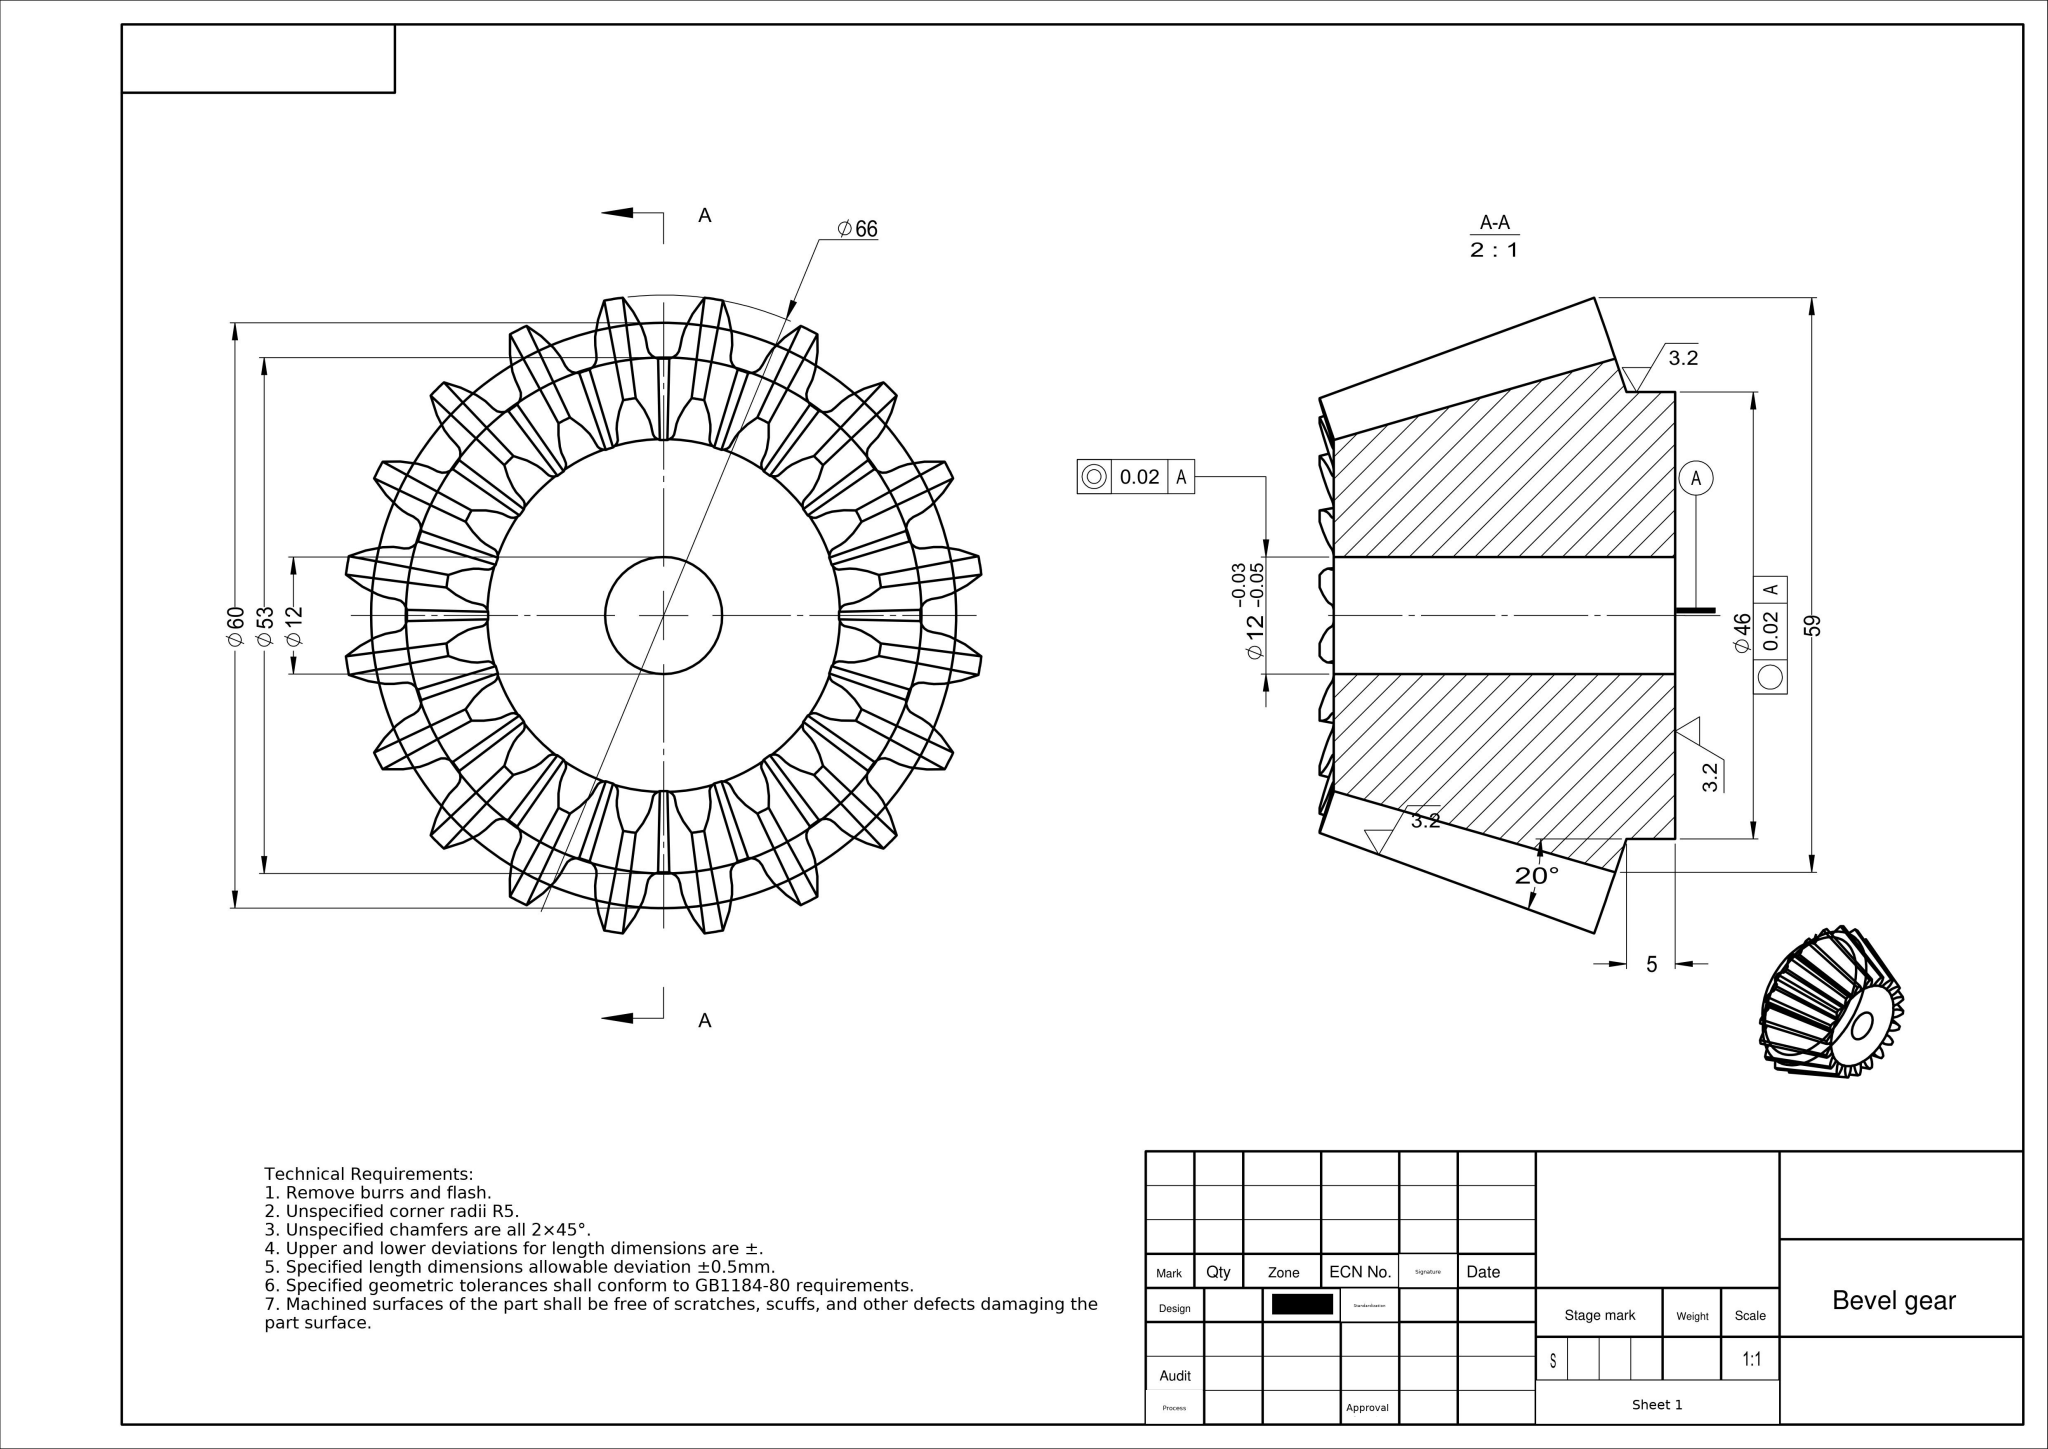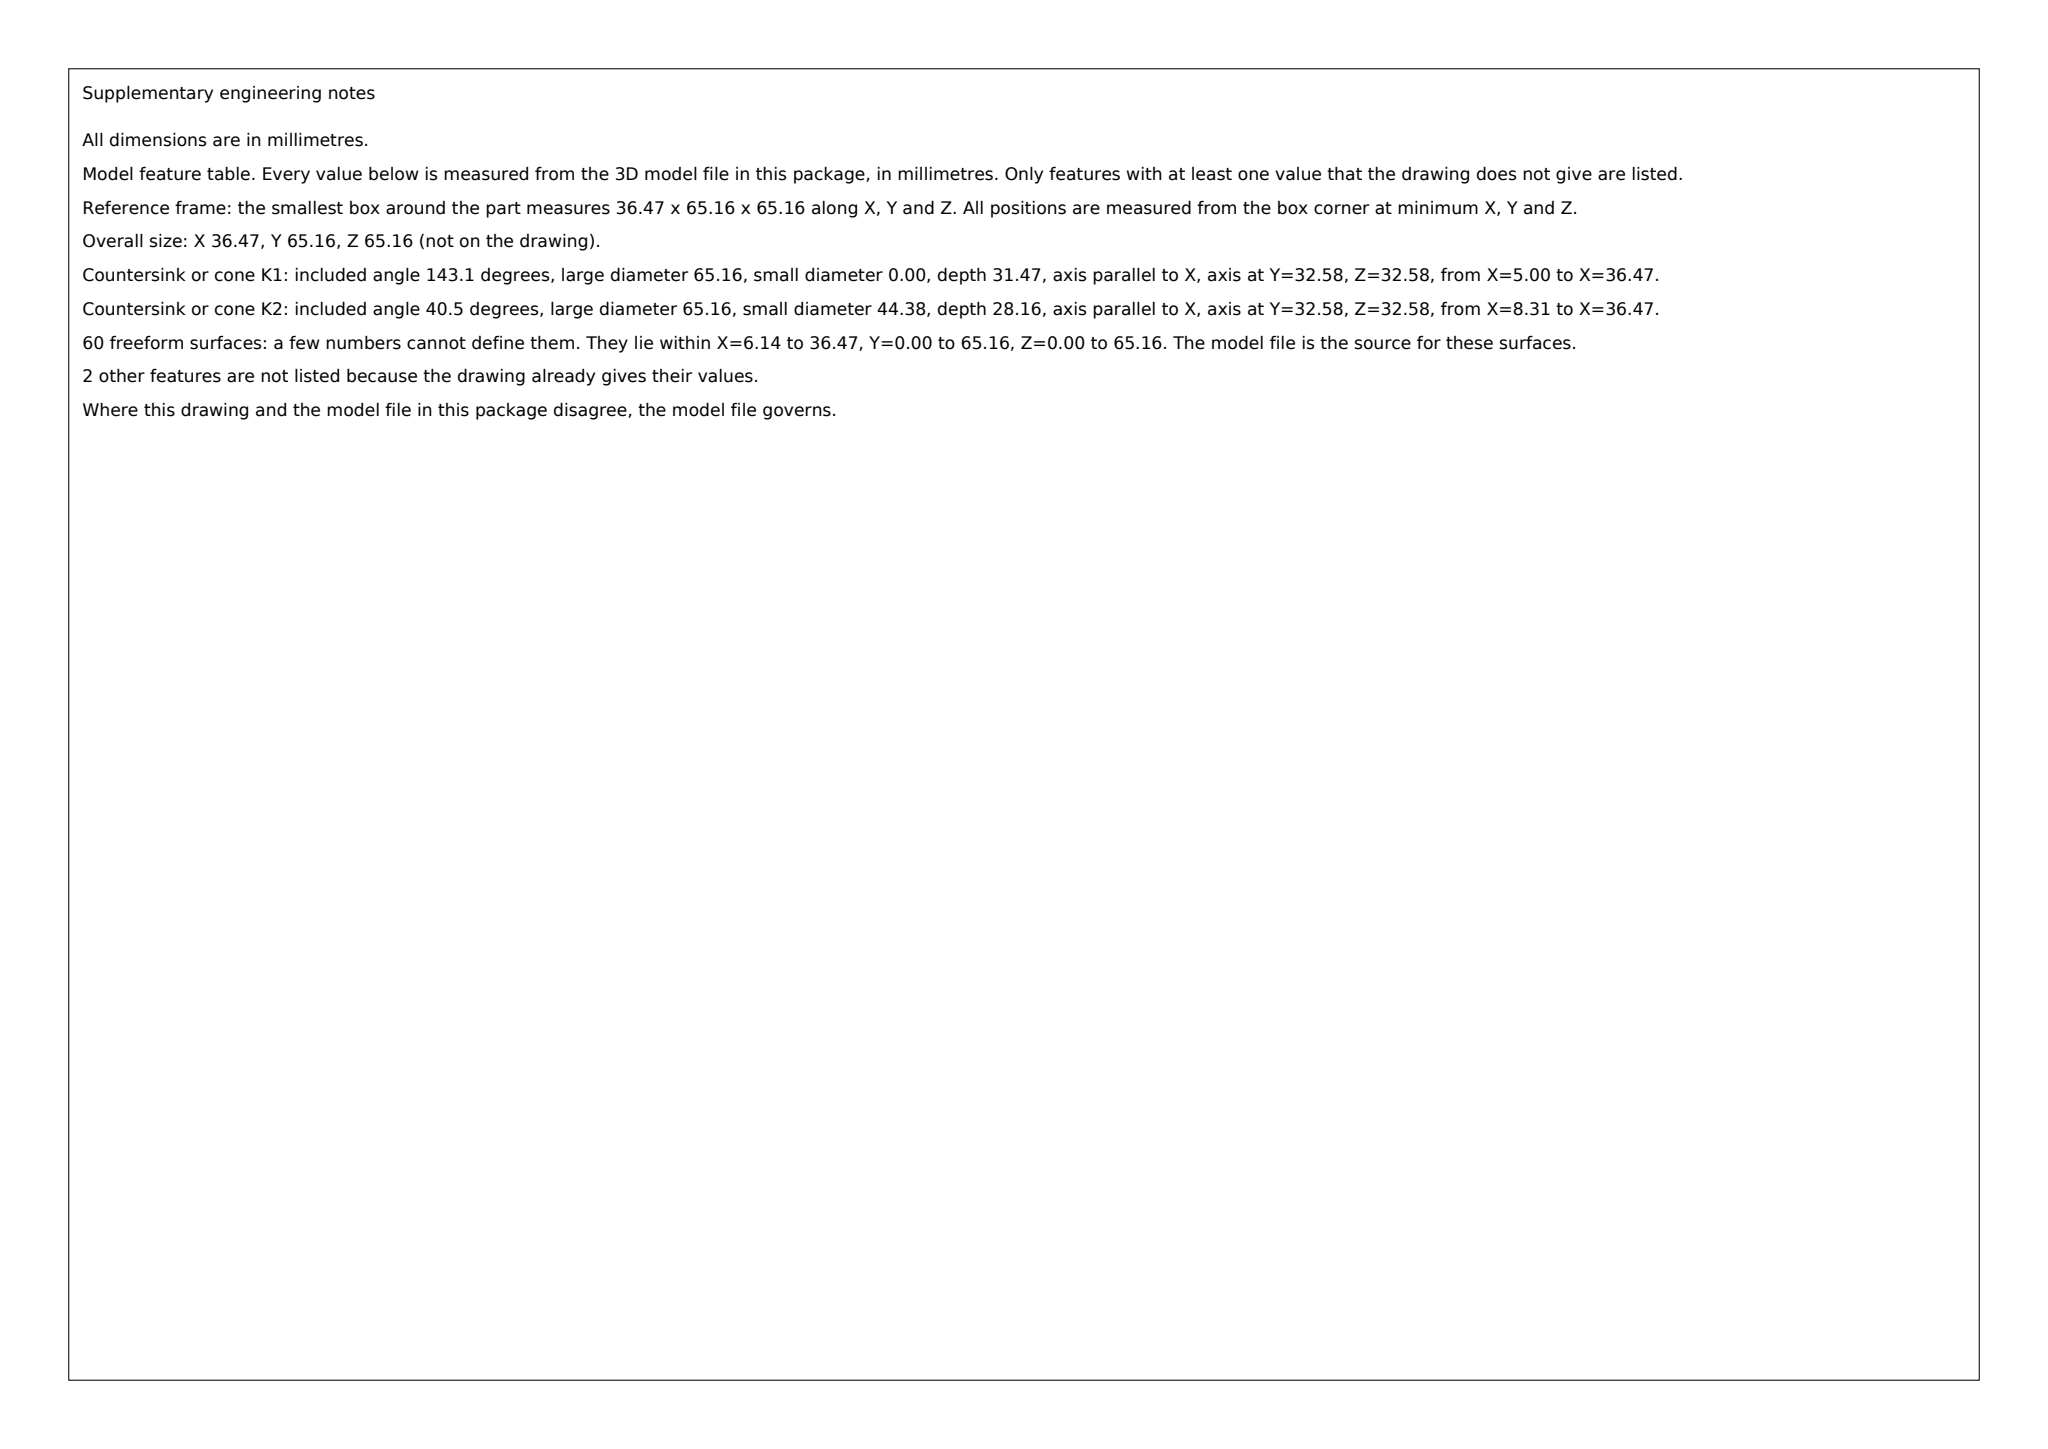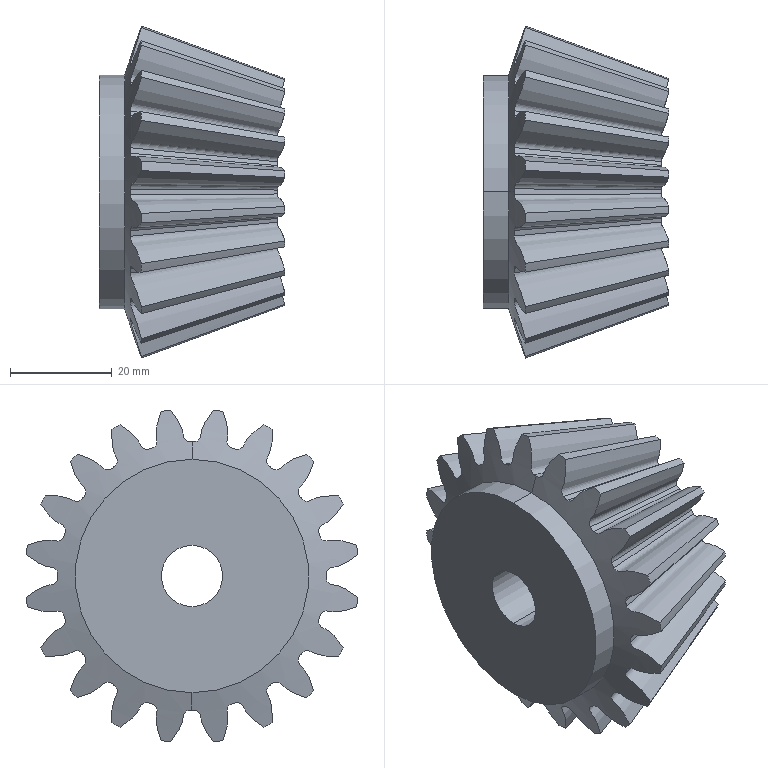Part | SolidWorks | mm | 1 solid | 108 faces | box 36.47 x 65.16 x 65.16 mm | volume 64692 mm3 | spline 60 | cone 42 | cylinder 4 | plane 2 | commonest cylinder face diameters 45.808 x2 12 x2